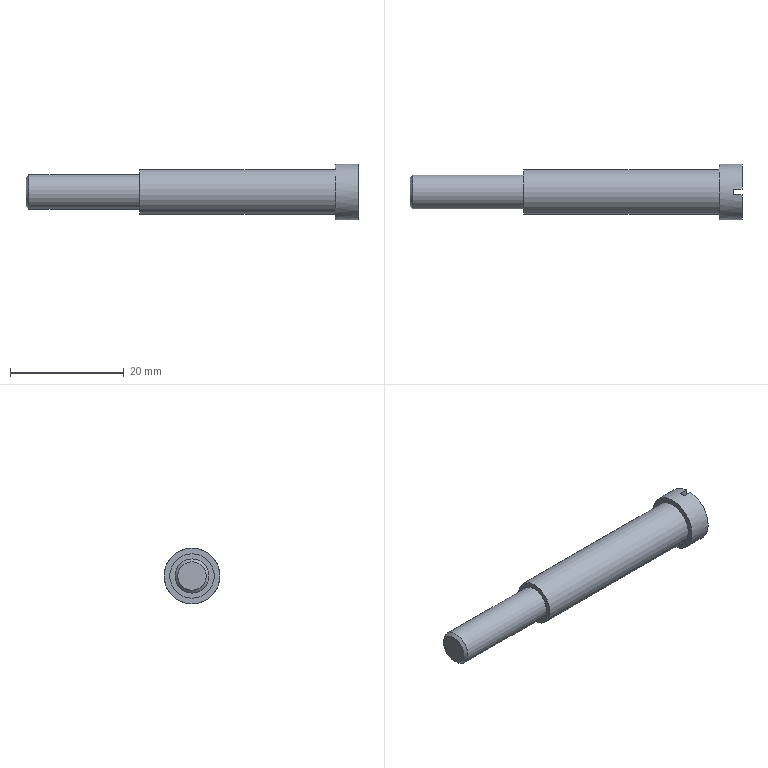Component | NX | HANDWHEEL_SHAFT_2 | 1 solid | 12 faces | box 58.4 x 9.8 x 9.8 mm | volume 2494 mm3 | plane 8 | cylinder 3 | cone 1 | commonest cylinder face diameters 9.8 x1 7.8 x1 6 x1
STEP:
#1=CARTESIAN_POINT('',(0.,0.,0.));
#2=DIRECTION('',(0.,0.,1.));
#3=DIRECTION('',(1.,0.,0.));
#4=AXIS2_PLACEMENT_3D('',#1,#2,#3);
#5=CARTESIAN_POINT('',(249.437,-20.232,106.126));
#6=VERTEX_POINT('',#5);
#7=CARTESIAN_POINT('',(249.437,-20.232,115.874));
#8=VERTEX_POINT('',#7);
#9=CARTESIAN_POINT('',(249.437,-19.732,111.));
#10=DIRECTION('',(-1.,0.,0.));
#11=DIRECTION('',(0.,0.,1.));
#12=AXIS2_PLACEMENT_3D('',#9,#10,#11);
#13=CIRCLE('',#12,4.9);
#14=CARTESIAN_POINT('',(249.437,-19.732,111.));
#15=DIRECTION('',(1.,0.,0.));
#16=DIRECTION('',(0.,0.,-1.));
#17=AXIS2_PLACEMENT_3D('',#14,#15,#16);
#18=PLANE('',#17);
#19=CARTESIAN_POINT('',(-4.9,0.));
#20=CARTESIAN_POINT('',(-4.9,8.487));
#21=CARTESIAN_POINT('',(2.45,4.244));
#22=CARTESIAN_POINT('',(9.8,0.));
#23=CARTESIAN_POINT('',(2.45,-4.244));
#24=CARTESIAN_POINT('',(-4.9,-8.487));
#25=CARTESIAN_POINT('',(-4.9,0.));
#26=(BOUNDED_CURVE()B_SPLINE_CURVE(2,(#19,#20,#21,#22,#23,#24,#25),.UNSPECIFIED.,.T.,.F.)B_SPLINE_CURVE_WITH_KNOTS((1,2,2,2,2,1),(-2.094,0.,2.094,4.189,6.283,8.378),.UNSPECIFIED.)CURVE()GEOMETRIC_REPRESENTATION_ITEM()RATIONAL_B_SPLINE_CURVE((1.,0.5,1.,0.5,1.,0.5,1.))REPRESENTATION_ITEM(''));
#27=(GEOMETRIC_REPRESENTATION_CONTEXT(2)PARAMETRIC_REPRESENTATION_CONTEXT()REPRESENTATION_CONTEXT('',''));
#28=DEFINITIONAL_REPRESENTATION('',(#26),#27);
#29=PCURVE('',#18,#28);
#30=CARTESIAN_POINT('',(249.437,-19.732,111.));
#31=DIRECTION('',(-1.,0.,0.));
#32=DIRECTION('',(0.,0.,1.));
#33=AXIS2_PLACEMENT_3D('',#30,#31,#32);
#34=CYLINDRICAL_SURFACE('',#33,4.9);
#35=CARTESIAN_POINT('',(0.,0.));
#36=DIRECTION('',(1.,0.));
#37=VECTOR('',#36,1.);
#38=LINE('',#35,#37);
#39=(GEOMETRIC_REPRESENTATION_CONTEXT(2)PARAMETRIC_REPRESENTATION_CONTEXT()REPRESENTATION_CONTEXT('',''));
#40=DEFINITIONAL_REPRESENTATION('',(#38),#39);
#41=PCURVE('',#34,#40);
#42=SURFACE_CURVE('',#13,(#29,#41),.PCURVE_S1.);
#43=EDGE_CURVE('',#6,#8,#42,.T.);
#44=ORIENTED_EDGE('',*,*,#43,.F.);
#45=CARTESIAN_POINT('',(249.437,-20.232,106.));
#46=DIRECTION('',(0.,0.,1.));
#47=VECTOR('',#46,1.);
#48=LINE('',#45,#47);
#49=CARTESIAN_POINT('',(5.,-0.5));
#50=DIRECTION('',(-1.,0.));
#51=VECTOR('',#50,1.);
#52=LINE('',#49,#51);
#53=(GEOMETRIC_REPRESENTATION_CONTEXT(2)PARAMETRIC_REPRESENTATION_CONTEXT()REPRESENTATION_CONTEXT('',''));
#54=DEFINITIONAL_REPRESENTATION('',(#52),#53);
#55=PCURVE('',#18,#54);
#56=CARTESIAN_POINT('',(249.437,-20.232,106.));
#57=DIRECTION('',(0.,-1.,0.));
#58=DIRECTION('',(1.,0.,0.));
#59=AXIS2_PLACEMENT_3D('',#56,#57,#58);
#60=PLANE('',#59);
#61=CARTESIAN_POINT('',(0.,0.));
#62=DIRECTION('',(0.,1.));
#63=VECTOR('',#62,1.);
#64=LINE('',#61,#63);
#65=(GEOMETRIC_REPRESENTATION_CONTEXT(2)PARAMETRIC_REPRESENTATION_CONTEXT()REPRESENTATION_CONTEXT('',''));
#66=DEFINITIONAL_REPRESENTATION('',(#64),#65);
#67=PCURVE('',#60,#66);
#68=SURFACE_CURVE('',#48,(#55,#67),.PCURVE_S1.);
#69=EDGE_CURVE('',#6,#8,#68,.T.);
#70=ORIENTED_EDGE('',*,*,#69,.T.);
#71=EDGE_LOOP('',(#44,#70));
#72=FACE_BOUND('',#71,.T.);
#73=ADVANCED_FACE('',(#72),#18,.T.);
#74=CARTESIAN_POINT('',(245.437,-19.732,114.9));
#75=VERTEX_POINT('',#74);
#76=CARTESIAN_POINT('',(245.437,-19.732,111.));
#77=DIRECTION('',(-1.,0.,0.));
#78=DIRECTION('',(0.,0.,1.));
#79=AXIS2_PLACEMENT_3D('',#76,#77,#78);
#80=CIRCLE('',#79,3.9);
#81=CARTESIAN_POINT('',(245.437,-19.732,111.));
#82=DIRECTION('',(-1.,0.,0.));
#83=DIRECTION('',(0.,0.,1.));
#84=AXIS2_PLACEMENT_3D('',#81,#82,#83);
#85=PLANE('',#84);
#86=CARTESIAN_POINT('',(0.,0.));
#87=DIRECTION('',(1.,0.));
#88=AXIS2_PLACEMENT_2D('',#86,#87);
#89=CIRCLE('',#88,3.9);
#90=(GEOMETRIC_REPRESENTATION_CONTEXT(2)PARAMETRIC_REPRESENTATION_CONTEXT()REPRESENTATION_CONTEXT('',''));
#91=DEFINITIONAL_REPRESENTATION('',(#89),#90);
#92=PCURVE('',#85,#91);
#93=CARTESIAN_POINT('',(245.437,-19.732,111.));
#94=DIRECTION('',(-1.,0.,0.));
#95=DIRECTION('',(0.,0.,1.));
#96=AXIS2_PLACEMENT_3D('',#93,#94,#95);
#97=CYLINDRICAL_SURFACE('',#96,3.9);
#98=CARTESIAN_POINT('',(0.,0.));
#99=DIRECTION('',(1.,0.));
#100=VECTOR('',#99,1.);
#101=LINE('',#98,#100);
#102=(GEOMETRIC_REPRESENTATION_CONTEXT(2)PARAMETRIC_REPRESENTATION_CONTEXT()REPRESENTATION_CONTEXT('',''));
#103=DEFINITIONAL_REPRESENTATION('',(#101),#102);
#104=PCURVE('',#97,#103);
#105=SURFACE_CURVE('',#80,(#92,#104),.PCURVE_S1.);
#106=EDGE_CURVE('',#75,#75,#105,.T.);
#107=ORIENTED_EDGE('',*,*,#106,.F.);
#108=EDGE_LOOP('',(#107));
#109=FACE_BOUND('',#108,.T.);
#110=CARTESIAN_POINT('',(245.437,-19.732,115.9));
#111=VERTEX_POINT('',#110);
#112=CARTESIAN_POINT('',(245.437,-19.732,111.));
#113=DIRECTION('',(1.,0.,0.));
#114=DIRECTION('',(0.,0.,1.));
#115=AXIS2_PLACEMENT_3D('',#112,#113,#114);
#116=CIRCLE('',#115,4.9);
#117=CARTESIAN_POINT('',(4.9,0.));
#118=CARTESIAN_POINT('',(4.9,-8.487));
#119=CARTESIAN_POINT('',(-2.45,-4.244));
#120=CARTESIAN_POINT('',(-9.8,-0.));
#121=CARTESIAN_POINT('',(-2.45,4.244));
#122=CARTESIAN_POINT('',(4.9,8.487));
#123=CARTESIAN_POINT('',(4.9,0.));
#124=(BOUNDED_CURVE()B_SPLINE_CURVE(2,(#117,#118,#119,#120,#121,#122,#123),.UNSPECIFIED.,.T.,.F.)B_SPLINE_CURVE_WITH_KNOTS((1,2,2,2,2,1),(-2.094,0.,2.094,4.189,6.283,8.378),.UNSPECIFIED.)CURVE()GEOMETRIC_REPRESENTATION_ITEM()RATIONAL_B_SPLINE_CURVE((1.,0.5,1.,0.5,1.,0.5,1.))REPRESENTATION_ITEM(''));
#125=(GEOMETRIC_REPRESENTATION_CONTEXT(2)PARAMETRIC_REPRESENTATION_CONTEXT()REPRESENTATION_CONTEXT('',''));
#126=DEFINITIONAL_REPRESENTATION('',(#124),#125);
#127=PCURVE('',#85,#126);
#128=CARTESIAN_POINT('',(6.283,4.));
#129=DIRECTION('',(-1.,0.));
#130=VECTOR('',#129,1.);
#131=LINE('',#128,#130);
#132=(GEOMETRIC_REPRESENTATION_CONTEXT(2)PARAMETRIC_REPRESENTATION_CONTEXT()REPRESENTATION_CONTEXT('',''));
#133=DEFINITIONAL_REPRESENTATION('',(#131),#132);
#134=PCURVE('',#34,#133);
#135=SURFACE_CURVE('',#116,(#127,#134),.PCURVE_S1.);
#136=EDGE_CURVE('',#111,#111,#135,.T.);
#137=ORIENTED_EDGE('',*,*,#136,.F.);
#138=EDGE_LOOP('',(#137));
#139=FACE_BOUND('',#138,.T.);
#140=ADVANCED_FACE('',(#109,#139),#85,.T.);
#141=CARTESIAN_POINT('',(249.437,-19.232,106.126));
#142=VERTEX_POINT('',#141);
#143=CARTESIAN_POINT('',(249.437,-19.232,115.874));
#144=VERTEX_POINT('',#143);
#145=CARTESIAN_POINT('',(249.437,-19.232,106.));
#146=DIRECTION('',(0.,0.,1.));
#147=VECTOR('',#146,1.);
#148=LINE('',#145,#147);
#149=CARTESIAN_POINT('',(249.437,-19.732,111.));
#150=DIRECTION('',(1.,0.,0.));
#151=DIRECTION('',(0.,0.,-1.));
#152=AXIS2_PLACEMENT_3D('',#149,#150,#151);
#153=PLANE('',#152);
#154=CARTESIAN_POINT('',(5.,0.5));
#155=DIRECTION('',(-1.,0.));
#156=VECTOR('',#155,1.);
#157=LINE('',#154,#156);
#158=(GEOMETRIC_REPRESENTATION_CONTEXT(2)PARAMETRIC_REPRESENTATION_CONTEXT()REPRESENTATION_CONTEXT('',''));
#159=DEFINITIONAL_REPRESENTATION('',(#157),#158);
#160=PCURVE('',#153,#159);
#161=CARTESIAN_POINT('',(249.437,-19.232,106.));
#162=DIRECTION('',(0.,-1.,0.));
#163=DIRECTION('',(1.,0.,0.));
#164=AXIS2_PLACEMENT_3D('',#161,#162,#163);
#165=PLANE('',#164);
#166=CARTESIAN_POINT('',(0.,0.));
#167=DIRECTION('',(0.,1.));
#168=VECTOR('',#167,1.);
#169=LINE('',#166,#168);
#170=(GEOMETRIC_REPRESENTATION_CONTEXT(2)PARAMETRIC_REPRESENTATION_CONTEXT()REPRESENTATION_CONTEXT('',''));
#171=DEFINITIONAL_REPRESENTATION('',(#169),#170);
#172=PCURVE('',#165,#171);
#173=SURFACE_CURVE('',#148,(#160,#172),.PCURVE_S1.);
#174=EDGE_CURVE('',#142,#144,#173,.T.);
#175=ORIENTED_EDGE('',*,*,#174,.F.);
#176=CARTESIAN_POINT('',(249.437,-19.732,111.));
#177=DIRECTION('',(-1.,0.,0.));
#178=DIRECTION('',(0.,0.,1.));
#179=AXIS2_PLACEMENT_3D('',#176,#177,#178);
#180=CIRCLE('',#179,4.9);
#181=CARTESIAN_POINT('',(-4.9,0.));
#182=CARTESIAN_POINT('',(-4.9,8.487));
#183=CARTESIAN_POINT('',(2.45,4.244));
#184=CARTESIAN_POINT('',(9.8,0.));
#185=CARTESIAN_POINT('',(2.45,-4.244));
#186=CARTESIAN_POINT('',(-4.9,-8.487));
#187=CARTESIAN_POINT('',(-4.9,0.));
#188=(BOUNDED_CURVE()B_SPLINE_CURVE(2,(#181,#182,#183,#184,#185,#186,#187),.UNSPECIFIED.,.T.,.F.)B_SPLINE_CURVE_WITH_KNOTS((1,2,2,2,2,1),(-2.094,0.,2.094,4.189,6.283,8.378),.UNSPECIFIED.)CURVE()GEOMETRIC_REPRESENTATION_ITEM()RATIONAL_B_SPLINE_CURVE((1.,0.5,1.,0.5,1.,0.5,1.))REPRESENTATION_ITEM(''));
#189=(GEOMETRIC_REPRESENTATION_CONTEXT(2)PARAMETRIC_REPRESENTATION_CONTEXT()REPRESENTATION_CONTEXT('',''));
#190=DEFINITIONAL_REPRESENTATION('',(#188),#189);
#191=PCURVE('',#153,#190);
#192=CARTESIAN_POINT('',(0.,0.));
#193=DIRECTION('',(1.,0.));
#194=VECTOR('',#193,1.);
#195=LINE('',#192,#194);
#196=(GEOMETRIC_REPRESENTATION_CONTEXT(2)PARAMETRIC_REPRESENTATION_CONTEXT()REPRESENTATION_CONTEXT('',''));
#197=DEFINITIONAL_REPRESENTATION('',(#195),#196);
#198=PCURVE('',#34,#197);
#199=SURFACE_CURVE('',#180,(#191,#198),.PCURVE_S1.);
#200=EDGE_CURVE('',#144,#142,#199,.T.);
#201=ORIENTED_EDGE('',*,*,#200,.F.);
#202=EDGE_LOOP('',(#175,#201));
#203=FACE_BOUND('',#202,.T.);
#204=ADVANCED_FACE('',(#203),#153,.T.);
#205=CARTESIAN_POINT('',(247.937,-20.232,115.874));
#206=VERTEX_POINT('',#205);
#207=CARTESIAN_POINT('',(249.437,-20.232,115.874));
#208=DIRECTION('',(1.,0.,0.));
#209=VECTOR('',#208,1.);
#210=LINE('',#207,#209);
#211=CARTESIAN_POINT('',(6.181,0.));
#212=DIRECTION('',(0.,-1.));
#213=VECTOR('',#212,1.);
#214=LINE('',#211,#213);
#215=(GEOMETRIC_REPRESENTATION_CONTEXT(2)PARAMETRIC_REPRESENTATION_CONTEXT()REPRESENTATION_CONTEXT('',''));
#216=DEFINITIONAL_REPRESENTATION('',(#214),#215);
#217=PCURVE('',#34,#216);
#218=CARTESIAN_POINT('',(0.,9.874));
#219=DIRECTION('',(1.,0.));
#220=VECTOR('',#219,1.);
#221=LINE('',#218,#220);
#222=(GEOMETRIC_REPRESENTATION_CONTEXT(2)PARAMETRIC_REPRESENTATION_CONTEXT()REPRESENTATION_CONTEXT('',''));
#223=DEFINITIONAL_REPRESENTATION('',(#221),#222);
#224=PCURVE('',#60,#223);
#225=SURFACE_CURVE('',#210,(#217,#224),.PCURVE_S1.);
#226=EDGE_CURVE('',#206,#8,#225,.T.);
#227=ORIENTED_EDGE('',*,*,#226,.F.);
#228=CARTESIAN_POINT('',(247.937,-19.732,115.9));
#229=VERTEX_POINT('',#228);
#230=CARTESIAN_POINT('',(247.937,-19.732,111.));
#231=DIRECTION('',(1.,0.,0.));
#232=DIRECTION('',(0.,0.,-1.));
#233=AXIS2_PLACEMENT_3D('',#230,#231,#232);
#234=CIRCLE('',#233,4.9);
#235=CARTESIAN_POINT('',(9.425,1.5));
#236=DIRECTION('',(-1.,0.));
#237=VECTOR('',#236,1.);
#238=LINE('',#235,#237);
#239=(GEOMETRIC_REPRESENTATION_CONTEXT(2)PARAMETRIC_REPRESENTATION_CONTEXT()REPRESENTATION_CONTEXT('',''));
#240=DEFINITIONAL_REPRESENTATION('',(#238),#239);
#241=PCURVE('',#34,#240);
#242=CARTESIAN_POINT('',(247.937,-19.732,106.));
#243=DIRECTION('',(1.,0.,0.));
#244=DIRECTION('',(0.,0.,1.));
#245=AXIS2_PLACEMENT_3D('',#242,#243,#244);
#246=PLANE('',#245);
#247=CARTESIAN_POINT('',(5.,0.));
#248=DIRECTION('',(-1.,0.));
#249=AXIS2_PLACEMENT_2D('',#247,#248);
#250=CIRCLE('',#249,4.9);
#251=(GEOMETRIC_REPRESENTATION_CONTEXT(2)PARAMETRIC_REPRESENTATION_CONTEXT()REPRESENTATION_CONTEXT('',''));
#252=DEFINITIONAL_REPRESENTATION('',(#250),#251);
#253=PCURVE('',#246,#252);
#254=SURFACE_CURVE('',#234,(#241,#253),.PCURVE_S1.);
#255=EDGE_CURVE('',#229,#206,#254,.T.);
#256=ORIENTED_EDGE('',*,*,#255,.F.);
#257=CARTESIAN_POINT('',(247.937,-19.732,115.9));
#258=CARTESIAN_POINT('',(245.437,-19.732,115.9));
#259=B_SPLINE_CURVE_WITH_KNOTS('',1,(#257,#258),.UNSPECIFIED.,.F.,.F.,(2,2),(1.5,4.),.PIECEWISE_BEZIER_KNOTS.);
#260=CARTESIAN_POINT('',(6.283,0.));
#261=DIRECTION('',(0.,1.));
#262=VECTOR('',#261,1.);
#263=LINE('',#260,#262);
#264=(GEOMETRIC_REPRESENTATION_CONTEXT(2)PARAMETRIC_REPRESENTATION_CONTEXT()REPRESENTATION_CONTEXT('',''));
#265=DEFINITIONAL_REPRESENTATION('',(#263),#264);
#266=PCURVE('',#34,#265);
#267=CARTESIAN_POINT('',(0.,0.));
#268=DIRECTION('',(0.,1.));
#269=VECTOR('',#268,1.);
#270=LINE('',#267,#269);
#271=(GEOMETRIC_REPRESENTATION_CONTEXT(2)PARAMETRIC_REPRESENTATION_CONTEXT()REPRESENTATION_CONTEXT('',''));
#272=DEFINITIONAL_REPRESENTATION('',(#270),#271);
#273=PCURVE('',#34,#272);
#274=SEAM_CURVE('',#259,(#266,#273),.PCURVE_S1.);
#275=EDGE_CURVE('',#229,#111,#274,.T.);
#276=ORIENTED_EDGE('',*,*,#275,.T.);
#277=ORIENTED_EDGE('',*,*,#136,.T.);
#278=ORIENTED_EDGE('',*,*,#275,.F.);
#279=CARTESIAN_POINT('',(247.937,-19.232,115.874));
#280=VERTEX_POINT('',#279);
#281=CARTESIAN_POINT('',(247.937,-19.732,111.));
#282=DIRECTION('',(1.,0.,0.));
#283=DIRECTION('',(0.,0.,-1.));
#284=AXIS2_PLACEMENT_3D('',#281,#282,#283);
#285=CIRCLE('',#284,4.9);
#286=CARTESIAN_POINT('',(3.142,1.5));
#287=DIRECTION('',(-1.,0.));
#288=VECTOR('',#287,1.);
#289=LINE('',#286,#288);
#290=(GEOMETRIC_REPRESENTATION_CONTEXT(2)PARAMETRIC_REPRESENTATION_CONTEXT()REPRESENTATION_CONTEXT('',''));
#291=DEFINITIONAL_REPRESENTATION('',(#289),#290);
#292=PCURVE('',#34,#291);
#293=CARTESIAN_POINT('',(5.,0.));
#294=DIRECTION('',(-1.,0.));
#295=AXIS2_PLACEMENT_2D('',#293,#294);
#296=CIRCLE('',#295,4.9);
#297=(GEOMETRIC_REPRESENTATION_CONTEXT(2)PARAMETRIC_REPRESENTATION_CONTEXT()REPRESENTATION_CONTEXT('',''));
#298=DEFINITIONAL_REPRESENTATION('',(#296),#297);
#299=PCURVE('',#246,#298);
#300=SURFACE_CURVE('',#285,(#292,#299),.PCURVE_S1.);
#301=EDGE_CURVE('',#280,#229,#300,.T.);
#302=ORIENTED_EDGE('',*,*,#301,.F.);
#303=CARTESIAN_POINT('',(249.437,-19.232,115.874));
#304=DIRECTION('',(1.,0.,0.));
#305=VECTOR('',#304,1.);
#306=LINE('',#303,#305);
#307=CARTESIAN_POINT('',(0.1022,0.));
#308=DIRECTION('',(0.,-1.));
#309=VECTOR('',#308,1.);
#310=LINE('',#307,#309);
#311=(GEOMETRIC_REPRESENTATION_CONTEXT(2)PARAMETRIC_REPRESENTATION_CONTEXT()REPRESENTATION_CONTEXT('',''));
#312=DEFINITIONAL_REPRESENTATION('',(#310),#311);
#313=PCURVE('',#34,#312);
#314=CARTESIAN_POINT('',(0.,9.874));
#315=DIRECTION('',(1.,0.));
#316=VECTOR('',#315,1.);
#317=LINE('',#314,#316);
#318=(GEOMETRIC_REPRESENTATION_CONTEXT(2)PARAMETRIC_REPRESENTATION_CONTEXT()REPRESENTATION_CONTEXT('',''));
#319=DEFINITIONAL_REPRESENTATION('',(#317),#318);
#320=PCURVE('',#165,#319);
#321=SURFACE_CURVE('',#306,(#313,#320),.PCURVE_S1.);
#322=EDGE_CURVE('',#280,#144,#321,.T.);
#323=ORIENTED_EDGE('',*,*,#322,.T.);
#324=ORIENTED_EDGE('',*,*,#200,.T.);
#325=CARTESIAN_POINT('',(247.937,-19.232,106.126));
#326=VERTEX_POINT('',#325);
#327=CARTESIAN_POINT('',(249.437,-19.232,106.126));
#328=DIRECTION('',(-1.,0.,0.));
#329=VECTOR('',#328,1.);
#330=LINE('',#327,#329);
#331=CARTESIAN_POINT('',(3.039,0.));
#332=DIRECTION('',(0.,1.));
#333=VECTOR('',#332,1.);
#334=LINE('',#331,#333);
#335=(GEOMETRIC_REPRESENTATION_CONTEXT(2)PARAMETRIC_REPRESENTATION_CONTEXT()REPRESENTATION_CONTEXT('',''));
#336=DEFINITIONAL_REPRESENTATION('',(#334),#335);
#337=PCURVE('',#34,#336);
#338=CARTESIAN_POINT('',(0.,0.1256));
#339=DIRECTION('',(-1.,0.));
#340=VECTOR('',#339,1.);
#341=LINE('',#338,#340);
#342=(GEOMETRIC_REPRESENTATION_CONTEXT(2)PARAMETRIC_REPRESENTATION_CONTEXT()REPRESENTATION_CONTEXT('',''));
#343=DEFINITIONAL_REPRESENTATION('',(#341),#342);
#344=PCURVE('',#165,#343);
#345=SURFACE_CURVE('',#330,(#337,#344),.PCURVE_S1.);
#346=EDGE_CURVE('',#142,#326,#345,.T.);
#347=ORIENTED_EDGE('',*,*,#346,.T.);
#348=CARTESIAN_POINT('',(247.937,-20.232,106.126));
#349=VERTEX_POINT('',#348);
#350=CARTESIAN_POINT('',(247.937,-19.732,111.));
#351=DIRECTION('',(1.,0.,0.));
#352=DIRECTION('',(0.,0.,-1.));
#353=AXIS2_PLACEMENT_3D('',#350,#351,#352);
#354=CIRCLE('',#353,4.9);
#355=CARTESIAN_POINT('',(9.425,1.5));
#356=DIRECTION('',(-1.,0.));
#357=VECTOR('',#356,1.);
#358=LINE('',#355,#357);
#359=(GEOMETRIC_REPRESENTATION_CONTEXT(2)PARAMETRIC_REPRESENTATION_CONTEXT()REPRESENTATION_CONTEXT('',''));
#360=DEFINITIONAL_REPRESENTATION('',(#358),#359);
#361=PCURVE('',#34,#360);
#362=CARTESIAN_POINT('',(5.,0.));
#363=DIRECTION('',(-1.,0.));
#364=AXIS2_PLACEMENT_2D('',#362,#363);
#365=CIRCLE('',#364,4.9);
#366=(GEOMETRIC_REPRESENTATION_CONTEXT(2)PARAMETRIC_REPRESENTATION_CONTEXT()REPRESENTATION_CONTEXT('',''));
#367=DEFINITIONAL_REPRESENTATION('',(#365),#366);
#368=PCURVE('',#246,#367);
#369=SURFACE_CURVE('',#354,(#361,#368),.PCURVE_S1.);
#370=EDGE_CURVE('',#349,#326,#369,.T.);
#371=ORIENTED_EDGE('',*,*,#370,.F.);
#372=CARTESIAN_POINT('',(249.437,-20.232,106.126));
#373=DIRECTION('',(-1.,0.,0.));
#374=VECTOR('',#373,1.);
#375=LINE('',#372,#374);
#376=CARTESIAN_POINT('',(3.244,0.));
#377=DIRECTION('',(0.,1.));
#378=VECTOR('',#377,1.);
#379=LINE('',#376,#378);
#380=(GEOMETRIC_REPRESENTATION_CONTEXT(2)PARAMETRIC_REPRESENTATION_CONTEXT()REPRESENTATION_CONTEXT('',''));
#381=DEFINITIONAL_REPRESENTATION('',(#379),#380);
#382=PCURVE('',#34,#381);
#383=CARTESIAN_POINT('',(0.,0.1256));
#384=DIRECTION('',(-1.,0.));
#385=VECTOR('',#384,1.);
#386=LINE('',#383,#385);
#387=(GEOMETRIC_REPRESENTATION_CONTEXT(2)PARAMETRIC_REPRESENTATION_CONTEXT()REPRESENTATION_CONTEXT('',''));
#388=DEFINITIONAL_REPRESENTATION('',(#386),#387);
#389=PCURVE('',#60,#388);
#390=SURFACE_CURVE('',#375,(#382,#389),.PCURVE_S1.);
#391=EDGE_CURVE('',#6,#349,#390,.T.);
#392=ORIENTED_EDGE('',*,*,#391,.F.);
#393=ORIENTED_EDGE('',*,*,#43,.T.);
#394=EDGE_LOOP('',(#227,#256,#276,#277,#278,#302,#323,#324,#347,#371,#392,#393));
#395=FACE_BOUND('',#394,.T.);
#396=ADVANCED_FACE('',(#395),#34,.T.);
#397=CARTESIAN_POINT('',(211.037,-19.732,114.));
#398=VERTEX_POINT('',#397);
#399=CARTESIAN_POINT('',(211.037,-19.732,111.));
#400=DIRECTION('',(-1.,0.,0.));
#401=DIRECTION('',(0.,0.,1.));
#402=AXIS2_PLACEMENT_3D('',#399,#400,#401);
#403=CIRCLE('',#402,3.);
#404=CARTESIAN_POINT('',(211.037,-19.732,111.));
#405=DIRECTION('',(-1.,0.,0.));
#406=DIRECTION('',(0.,0.,1.));
#407=AXIS2_PLACEMENT_3D('',#404,#405,#406);
#408=PLANE('',#407);
#409=CARTESIAN_POINT('',(0.,0.));
#410=DIRECTION('',(1.,0.));
#411=AXIS2_PLACEMENT_2D('',#409,#410);
#412=CIRCLE('',#411,3.);
#413=(GEOMETRIC_REPRESENTATION_CONTEXT(2)PARAMETRIC_REPRESENTATION_CONTEXT()REPRESENTATION_CONTEXT('',''));
#414=DEFINITIONAL_REPRESENTATION('',(#412),#413);
#415=PCURVE('',#408,#414);
#416=CARTESIAN_POINT('',(211.037,-19.732,111.));
#417=DIRECTION('',(-1.,0.,0.));
#418=DIRECTION('',(0.,0.,1.));
#419=AXIS2_PLACEMENT_3D('',#416,#417,#418);
#420=CYLINDRICAL_SURFACE('',#419,3.);
#421=CARTESIAN_POINT('',(0.,0.));
#422=DIRECTION('',(1.,0.));
#423=VECTOR('',#422,1.);
#424=LINE('',#421,#423);
#425=(GEOMETRIC_REPRESENTATION_CONTEXT(2)PARAMETRIC_REPRESENTATION_CONTEXT()REPRESENTATION_CONTEXT('',''));
#426=DEFINITIONAL_REPRESENTATION('',(#424),#425);
#427=PCURVE('',#420,#426);
#428=SURFACE_CURVE('',#403,(#415,#427),.PCURVE_S1.);
#429=EDGE_CURVE('',#398,#398,#428,.T.);
#430=ORIENTED_EDGE('',*,*,#429,.F.);
#431=EDGE_LOOP('',(#430));
#432=FACE_BOUND('',#431,.T.);
#433=CARTESIAN_POINT('',(211.037,-19.732,114.9));
#434=VERTEX_POINT('',#433);
#435=CARTESIAN_POINT('',(211.037,-19.732,111.));
#436=DIRECTION('',(1.,0.,0.));
#437=DIRECTION('',(0.,0.,1.));
#438=AXIS2_PLACEMENT_3D('',#435,#436,#437);
#439=CIRCLE('',#438,3.9);
#440=CARTESIAN_POINT('',(3.9,0.));
#441=CARTESIAN_POINT('',(3.9,-6.755));
#442=CARTESIAN_POINT('',(-1.95,-3.377));
#443=CARTESIAN_POINT('',(-7.8,-0.));
#444=CARTESIAN_POINT('',(-1.95,3.377));
#445=CARTESIAN_POINT('',(3.9,6.755));
#446=CARTESIAN_POINT('',(3.9,0.));
#447=(BOUNDED_CURVE()B_SPLINE_CURVE(2,(#440,#441,#442,#443,#444,#445,#446),.UNSPECIFIED.,.T.,.F.)B_SPLINE_CURVE_WITH_KNOTS((1,2,2,2,2,1),(-2.094,0.,2.094,4.189,6.283,8.378),.UNSPECIFIED.)CURVE()GEOMETRIC_REPRESENTATION_ITEM()RATIONAL_B_SPLINE_CURVE((1.,0.5,1.,0.5,1.,0.5,1.))REPRESENTATION_ITEM(''));
#448=(GEOMETRIC_REPRESENTATION_CONTEXT(2)PARAMETRIC_REPRESENTATION_CONTEXT()REPRESENTATION_CONTEXT('',''));
#449=DEFINITIONAL_REPRESENTATION('',(#447),#448);
#450=PCURVE('',#408,#449);
#451=CARTESIAN_POINT('',(6.283,34.4));
#452=DIRECTION('',(-1.,0.));
#453=VECTOR('',#452,1.);
#454=LINE('',#451,#453);
#455=(GEOMETRIC_REPRESENTATION_CONTEXT(2)PARAMETRIC_REPRESENTATION_CONTEXT()REPRESENTATION_CONTEXT('',''));
#456=DEFINITIONAL_REPRESENTATION('',(#454),#455);
#457=PCURVE('',#97,#456);
#458=SURFACE_CURVE('',#439,(#450,#457),.PCURVE_S1.);
#459=EDGE_CURVE('',#434,#434,#458,.T.);
#460=ORIENTED_EDGE('',*,*,#459,.F.);
#461=EDGE_LOOP('',(#460));
#462=FACE_BOUND('',#461,.T.);
#463=ADVANCED_FACE('',(#432,#462),#408,.T.);
#464=ORIENTED_EDGE('',*,*,#459,.T.);
#465=CARTESIAN_POINT('',(245.437,-19.732,114.9));
#466=CARTESIAN_POINT('',(211.037,-19.732,114.9));
#467=B_SPLINE_CURVE_WITH_KNOTS('',1,(#465,#466),.UNSPECIFIED.,.F.,.F.,(2,2),(0.,34.4),.PIECEWISE_BEZIER_KNOTS.);
#468=CARTESIAN_POINT('',(0.,0.));
#469=DIRECTION('',(0.,1.));
#470=VECTOR('',#469,1.);
#471=LINE('',#468,#470);
#472=(GEOMETRIC_REPRESENTATION_CONTEXT(2)PARAMETRIC_REPRESENTATION_CONTEXT()REPRESENTATION_CONTEXT('',''));
#473=DEFINITIONAL_REPRESENTATION('',(#471),#472);
#474=PCURVE('',#97,#473);
#475=CARTESIAN_POINT('',(6.283,0.));
#476=DIRECTION('',(0.,1.));
#477=VECTOR('',#476,1.);
#478=LINE('',#475,#477);
#479=(GEOMETRIC_REPRESENTATION_CONTEXT(2)PARAMETRIC_REPRESENTATION_CONTEXT()REPRESENTATION_CONTEXT('',''));
#480=DEFINITIONAL_REPRESENTATION('',(#478),#479);
#481=PCURVE('',#97,#480);
#482=SEAM_CURVE('',#467,(#474,#481),.PCURVE_S1.);
#483=EDGE_CURVE('',#75,#434,#482,.T.);
#484=ORIENTED_EDGE('',*,*,#483,.F.);
#485=ORIENTED_EDGE('',*,*,#106,.T.);
#486=ORIENTED_EDGE('',*,*,#483,.T.);
#487=EDGE_LOOP('',(#464,#484,#485,#486));
#488=FACE_BOUND('',#487,.T.);
#489=ADVANCED_FACE('',(#488),#97,.T.);
#490=CARTESIAN_POINT('',(191.037,-19.732,113.5));
#491=VERTEX_POINT('',#490);
#492=CARTESIAN_POINT('',(191.037,-19.732,111.));
#493=DIRECTION('',(-1.,0.,0.));
#494=DIRECTION('',(0.,0.,1.));
#495=AXIS2_PLACEMENT_3D('',#492,#493,#494);
#496=CIRCLE('',#495,2.5);
#497=CARTESIAN_POINT('',(191.037,-19.732,111.));
#498=DIRECTION('',(-1.,0.,0.));
#499=DIRECTION('',(0.,0.,1.));
#500=AXIS2_PLACEMENT_3D('',#497,#498,#499);
#501=PLANE('',#500);
#502=CARTESIAN_POINT('',(0.,0.));
#503=DIRECTION('',(1.,0.));
#504=AXIS2_PLACEMENT_2D('',#502,#503);
#505=CIRCLE('',#504,2.5);
#506=(GEOMETRIC_REPRESENTATION_CONTEXT(2)PARAMETRIC_REPRESENTATION_CONTEXT()REPRESENTATION_CONTEXT('',''));
#507=DEFINITIONAL_REPRESENTATION('',(#505),#506);
#508=PCURVE('',#501,#507);
#509=CARTESIAN_POINT('',(191.537,-19.732,111.));
#510=DIRECTION('',(1.,0.,0.));
#511=DIRECTION('',(0.,0.,-1.));
#512=AXIS2_PLACEMENT_3D('',#509,#510,#511);
#513=CONICAL_SURFACE('',#512,3.,0.7854);
#514=CARTESIAN_POINT('',(9.425,-0.5));
#515=DIRECTION('',(-1.,0.));
#516=VECTOR('',#515,1.);
#517=LINE('',#514,#516);
#518=(GEOMETRIC_REPRESENTATION_CONTEXT(2)PARAMETRIC_REPRESENTATION_CONTEXT()REPRESENTATION_CONTEXT('',''));
#519=DEFINITIONAL_REPRESENTATION('',(#517),#518);
#520=PCURVE('',#513,#519);
#521=SURFACE_CURVE('',#496,(#508,#520),.PCURVE_S1.);
#522=EDGE_CURVE('',#491,#491,#521,.T.);
#523=ORIENTED_EDGE('',*,*,#522,.T.);
#524=EDGE_LOOP('',(#523));
#525=FACE_BOUND('',#524,.T.);
#526=ADVANCED_FACE('',(#525),#501,.T.);
#527=CARTESIAN_POINT('',(191.537,-19.732,114.));
#528=VERTEX_POINT('',#527);
#529=CARTESIAN_POINT('',(191.537,-19.732,111.));
#530=DIRECTION('',(1.,0.,0.));
#531=DIRECTION('',(0.,0.,1.));
#532=AXIS2_PLACEMENT_3D('',#529,#530,#531);
#533=CIRCLE('',#532,3.);
#534=CARTESIAN_POINT('',(6.283,19.5));
#535=DIRECTION('',(-1.,0.));
#536=VECTOR('',#535,1.);
#537=LINE('',#534,#536);
#538=(GEOMETRIC_REPRESENTATION_CONTEXT(2)PARAMETRIC_REPRESENTATION_CONTEXT()REPRESENTATION_CONTEXT('',''));
#539=DEFINITIONAL_REPRESENTATION('',(#537),#538);
#540=PCURVE('',#420,#539);
#541=CARTESIAN_POINT('',(3.142,0.));
#542=DIRECTION('',(1.,0.));
#543=VECTOR('',#542,1.);
#544=LINE('',#541,#543);
#545=(GEOMETRIC_REPRESENTATION_CONTEXT(2)PARAMETRIC_REPRESENTATION_CONTEXT()REPRESENTATION_CONTEXT('',''));
#546=DEFINITIONAL_REPRESENTATION('',(#544),#545);
#547=PCURVE('',#513,#546);
#548=SURFACE_CURVE('',#533,(#540,#547),.PCURVE_S1.);
#549=EDGE_CURVE('',#528,#528,#548,.T.);
#550=ORIENTED_EDGE('',*,*,#549,.T.);
#551=CARTESIAN_POINT('',(211.037,-19.732,114.));
#552=CARTESIAN_POINT('',(191.537,-19.732,114.));
#553=B_SPLINE_CURVE_WITH_KNOTS('',1,(#551,#552),.UNSPECIFIED.,.F.,.F.,(2,2),(0.,19.5),.PIECEWISE_BEZIER_KNOTS.);
#554=CARTESIAN_POINT('',(0.,0.));
#555=DIRECTION('',(0.,1.));
#556=VECTOR('',#555,1.);
#557=LINE('',#554,#556);
#558=(GEOMETRIC_REPRESENTATION_CONTEXT(2)PARAMETRIC_REPRESENTATION_CONTEXT()REPRESENTATION_CONTEXT('',''));
#559=DEFINITIONAL_REPRESENTATION('',(#557),#558);
#560=PCURVE('',#420,#559);
#561=CARTESIAN_POINT('',(6.283,0.));
#562=DIRECTION('',(0.,1.));
#563=VECTOR('',#562,1.);
#564=LINE('',#561,#563);
#565=(GEOMETRIC_REPRESENTATION_CONTEXT(2)PARAMETRIC_REPRESENTATION_CONTEXT()REPRESENTATION_CONTEXT('',''));
#566=DEFINITIONAL_REPRESENTATION('',(#564),#565);
#567=PCURVE('',#420,#566);
#568=SEAM_CURVE('',#553,(#560,#567),.PCURVE_S1.);
#569=EDGE_CURVE('',#398,#528,#568,.T.);
#570=ORIENTED_EDGE('',*,*,#569,.F.);
#571=ORIENTED_EDGE('',*,*,#429,.T.);
#572=ORIENTED_EDGE('',*,*,#569,.T.);
#573=EDGE_LOOP('',(#550,#570,#571,#572));
#574=FACE_BOUND('',#573,.T.);
#575=ADVANCED_FACE('',(#574),#420,.T.);
#576=ORIENTED_EDGE('',*,*,#522,.F.);
#577=CARTESIAN_POINT('',(191.037,-19.732,113.5));
#578=CARTESIAN_POINT('',(191.537,-19.732,114.));
#579=B_SPLINE_CURVE_WITH_KNOTS('',1,(#577,#578),.UNSPECIFIED.,.F.,.F.,(2,2),(-0.7071,0.),.PIECEWISE_BEZIER_KNOTS.);
#580=CARTESIAN_POINT('',(9.425,0.));
#581=DIRECTION('',(0.,1.));
#582=VECTOR('',#581,1.);
#583=LINE('',#580,#582);
#584=(GEOMETRIC_REPRESENTATION_CONTEXT(2)PARAMETRIC_REPRESENTATION_CONTEXT()REPRESENTATION_CONTEXT('',''));
#585=DEFINITIONAL_REPRESENTATION('',(#583),#584);
#586=PCURVE('',#513,#585);
#587=CARTESIAN_POINT('',(3.142,0.));
#588=DIRECTION('',(0.,1.));
#589=VECTOR('',#588,1.);
#590=LINE('',#587,#589);
#591=(GEOMETRIC_REPRESENTATION_CONTEXT(2)PARAMETRIC_REPRESENTATION_CONTEXT()REPRESENTATION_CONTEXT('',''));
#592=DEFINITIONAL_REPRESENTATION('',(#590),#591);
#593=PCURVE('',#513,#592);
#594=SEAM_CURVE('',#579,(#586,#593),.PCURVE_S1.);
#595=EDGE_CURVE('',#491,#528,#594,.T.);
#596=ORIENTED_EDGE('',*,*,#595,.T.);
#597=ORIENTED_EDGE('',*,*,#549,.F.);
#598=ORIENTED_EDGE('',*,*,#595,.F.);
#599=EDGE_LOOP('',(#576,#596,#597,#598));
#600=FACE_BOUND('',#599,.T.);
#601=ADVANCED_FACE('',(#600),#513,.T.);
#602=ORIENTED_EDGE('',*,*,#301,.T.);
#603=ORIENTED_EDGE('',*,*,#255,.T.);
#604=CARTESIAN_POINT('',(247.937,-20.232,106.));
#605=DIRECTION('',(0.,0.,-1.));
#606=VECTOR('',#605,1.);
#607=LINE('',#604,#606);
#608=CARTESIAN_POINT('',(0.,0.5));
#609=DIRECTION('',(-1.,0.));
#610=VECTOR('',#609,1.);
#611=LINE('',#608,#610);
#612=(GEOMETRIC_REPRESENTATION_CONTEXT(2)PARAMETRIC_REPRESENTATION_CONTEXT()REPRESENTATION_CONTEXT('',''));
#613=DEFINITIONAL_REPRESENTATION('',(#611),#612);
#614=PCURVE('',#246,#613);
#615=CARTESIAN_POINT('',(-1.5,0.));
#616=DIRECTION('',(0.,-1.));
#617=VECTOR('',#616,1.);
#618=LINE('',#615,#617);
#619=(GEOMETRIC_REPRESENTATION_CONTEXT(2)PARAMETRIC_REPRESENTATION_CONTEXT()REPRESENTATION_CONTEXT('',''));
#620=DEFINITIONAL_REPRESENTATION('',(#618),#619);
#621=PCURVE('',#60,#620);
#622=SURFACE_CURVE('',#607,(#614,#621),.PCURVE_S1.);
#623=EDGE_CURVE('',#206,#349,#622,.T.);
#624=ORIENTED_EDGE('',*,*,#623,.T.);
#625=ORIENTED_EDGE('',*,*,#370,.T.);
#626=CARTESIAN_POINT('',(247.937,-19.232,106.));
#627=DIRECTION('',(0.,0.,-1.));
#628=VECTOR('',#627,1.);
#629=LINE('',#626,#628);
#630=CARTESIAN_POINT('',(0.,-0.5));
#631=DIRECTION('',(-1.,0.));
#632=VECTOR('',#631,1.);
#633=LINE('',#630,#632);
#634=(GEOMETRIC_REPRESENTATION_CONTEXT(2)PARAMETRIC_REPRESENTATION_CONTEXT()REPRESENTATION_CONTEXT('',''));
#635=DEFINITIONAL_REPRESENTATION('',(#633),#634);
#636=PCURVE('',#246,#635);
#637=CARTESIAN_POINT('',(-1.5,0.));
#638=DIRECTION('',(0.,-1.));
#639=VECTOR('',#638,1.);
#640=LINE('',#637,#639);
#641=(GEOMETRIC_REPRESENTATION_CONTEXT(2)PARAMETRIC_REPRESENTATION_CONTEXT()REPRESENTATION_CONTEXT('',''));
#642=DEFINITIONAL_REPRESENTATION('',(#640),#641);
#643=PCURVE('',#165,#642);
#644=SURFACE_CURVE('',#629,(#636,#643),.PCURVE_S1.);
#645=EDGE_CURVE('',#280,#326,#644,.T.);
#646=ORIENTED_EDGE('',*,*,#645,.F.);
#647=EDGE_LOOP('',(#602,#603,#624,#625,#646));
#648=FACE_BOUND('',#647,.T.);
#649=ADVANCED_FACE('',(#648),#246,.T.);
#650=ORIENTED_EDGE('',*,*,#226,.T.);
#651=ORIENTED_EDGE('',*,*,#69,.F.);
#652=ORIENTED_EDGE('',*,*,#391,.T.);
#653=ORIENTED_EDGE('',*,*,#623,.F.);
#654=EDGE_LOOP('',(#650,#651,#652,#653));
#655=FACE_BOUND('',#654,.T.);
#656=ADVANCED_FACE('',(#655),#60,.F.);
#657=ORIENTED_EDGE('',*,*,#645,.T.);
#658=ORIENTED_EDGE('',*,*,#346,.F.);
#659=ORIENTED_EDGE('',*,*,#174,.T.);
#660=ORIENTED_EDGE('',*,*,#322,.F.);
#661=EDGE_LOOP('',(#657,#658,#659,#660));
#662=FACE_BOUND('',#661,.T.);
#663=ADVANCED_FACE('',(#662),#165,.T.);
#664=CLOSED_SHELL('',(#73,#140,#204,#396,#463,#489,#526,#575,#601,#649,#656,#663));
#665=MANIFOLD_SOLID_BREP('',#664);
#666=(LENGTH_UNIT()NAMED_UNIT(*)SI_UNIT(.MILLI.,.METRE.));
#667=UNCERTAINTY_MEASURE_WITH_UNIT(LENGTH_MEASURE(0.000005),#666,'','');
#668=(NAMED_UNIT(*)PLANE_ANGLE_UNIT()SI_UNIT($,.RADIAN.));
#669=(NAMED_UNIT(*)SI_UNIT($,.STERADIAN.)SOLID_ANGLE_UNIT());
#670=(GEOMETRIC_REPRESENTATION_CONTEXT(3)GLOBAL_UNCERTAINTY_ASSIGNED_CONTEXT((#667))GLOBAL_UNIT_ASSIGNED_CONTEXT((#666,#668,#669))REPRESENTATION_CONTEXT('',''));
#671=ADVANCED_BREP_SHAPE_REPRESENTATION('',(#4,#665),#670);